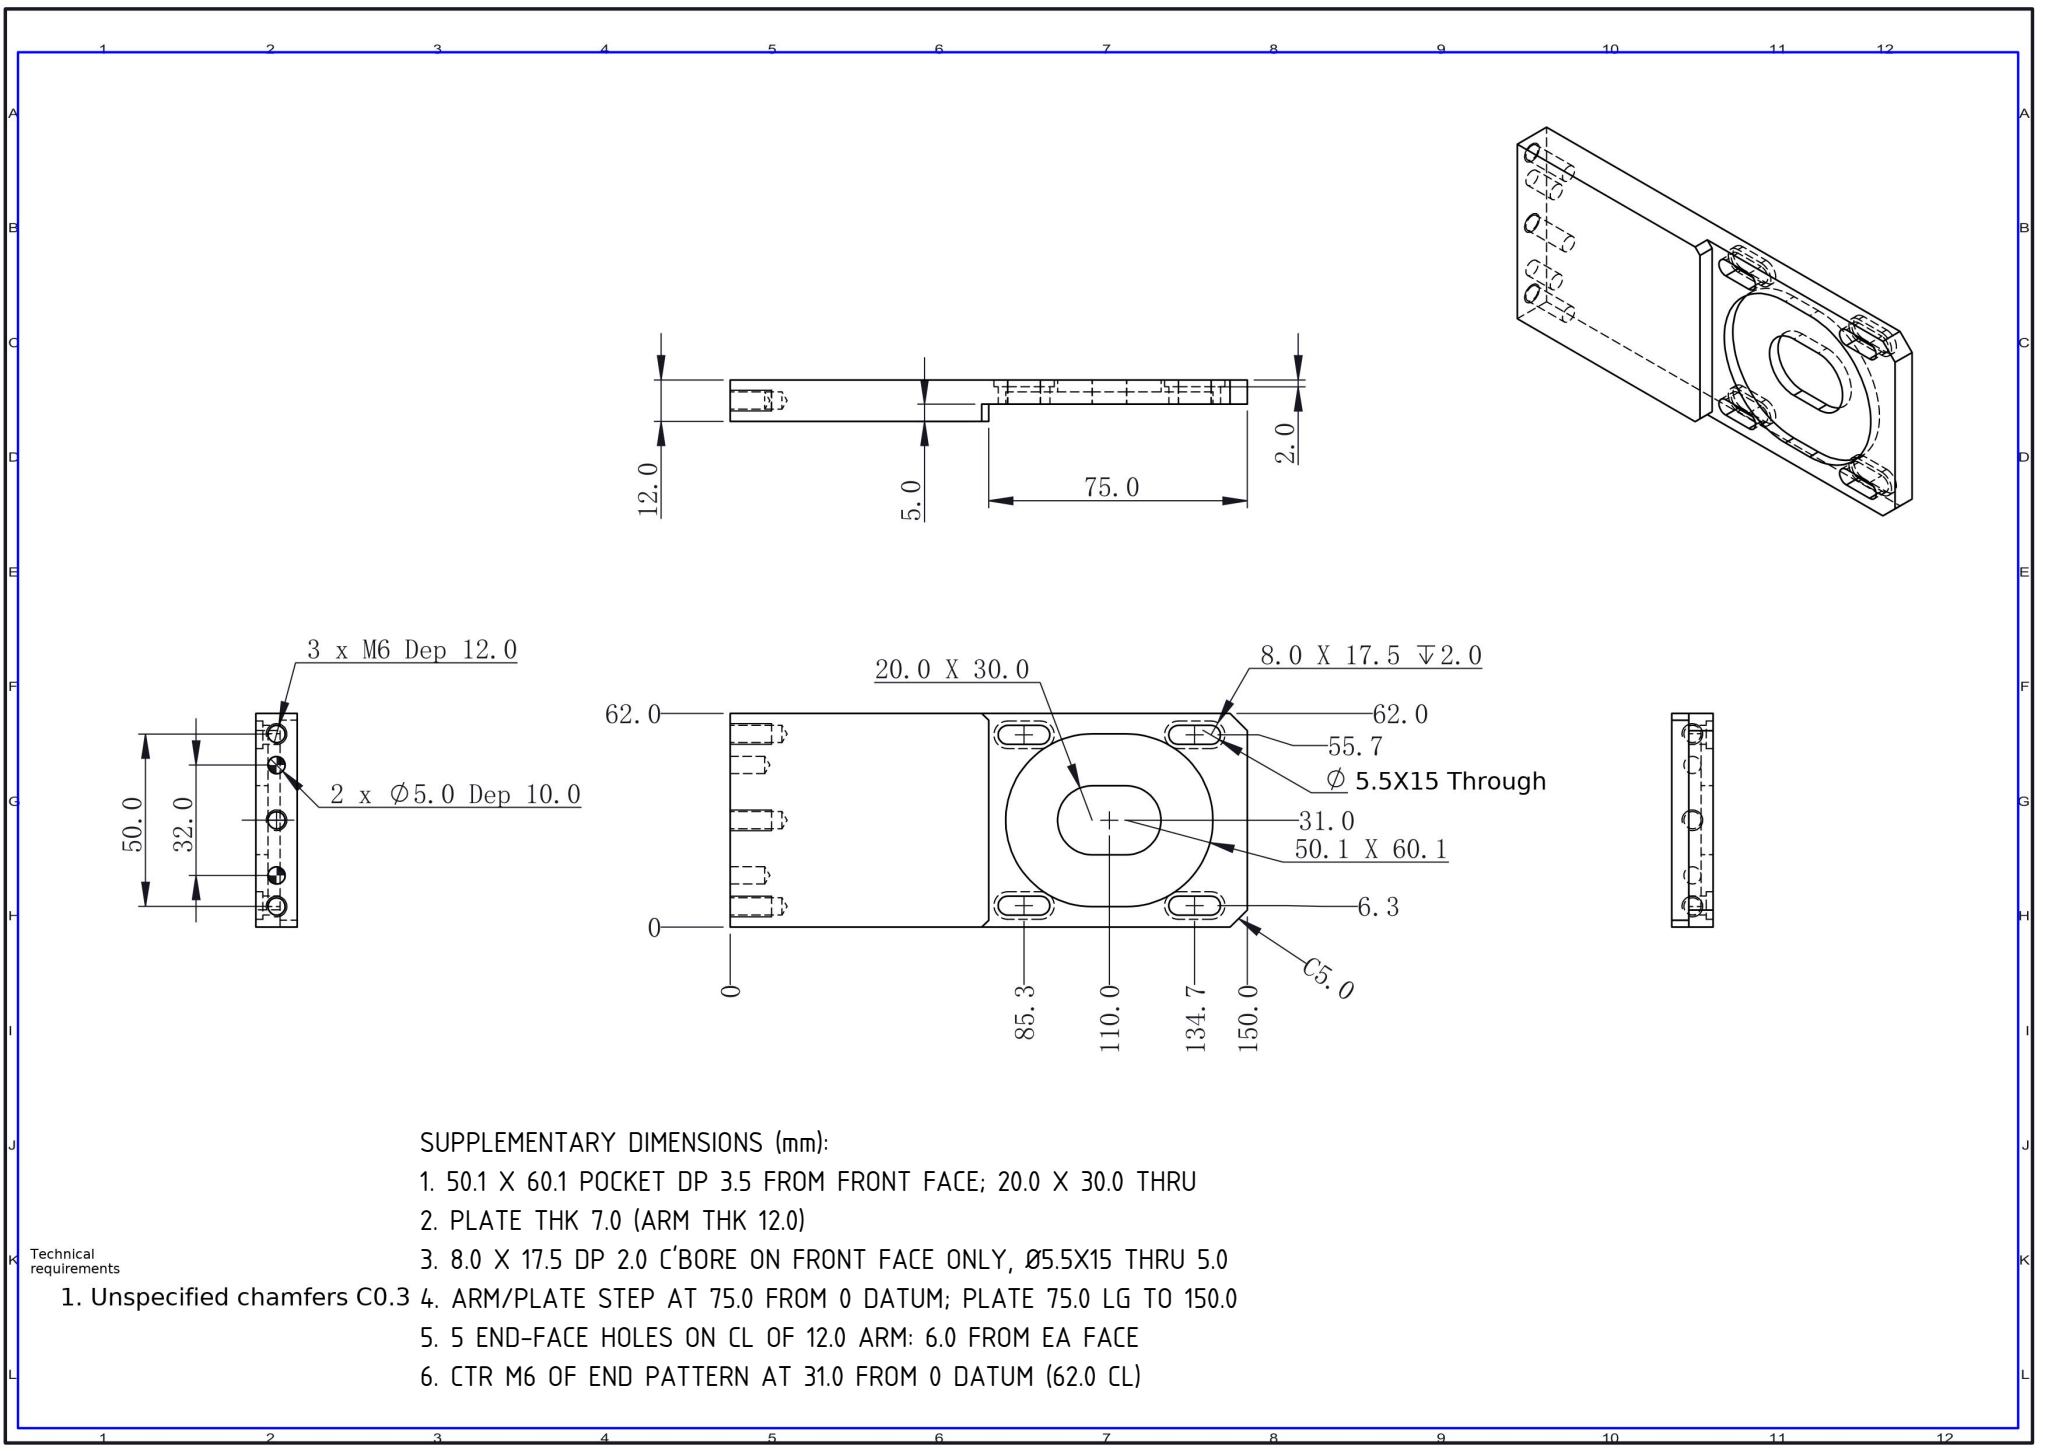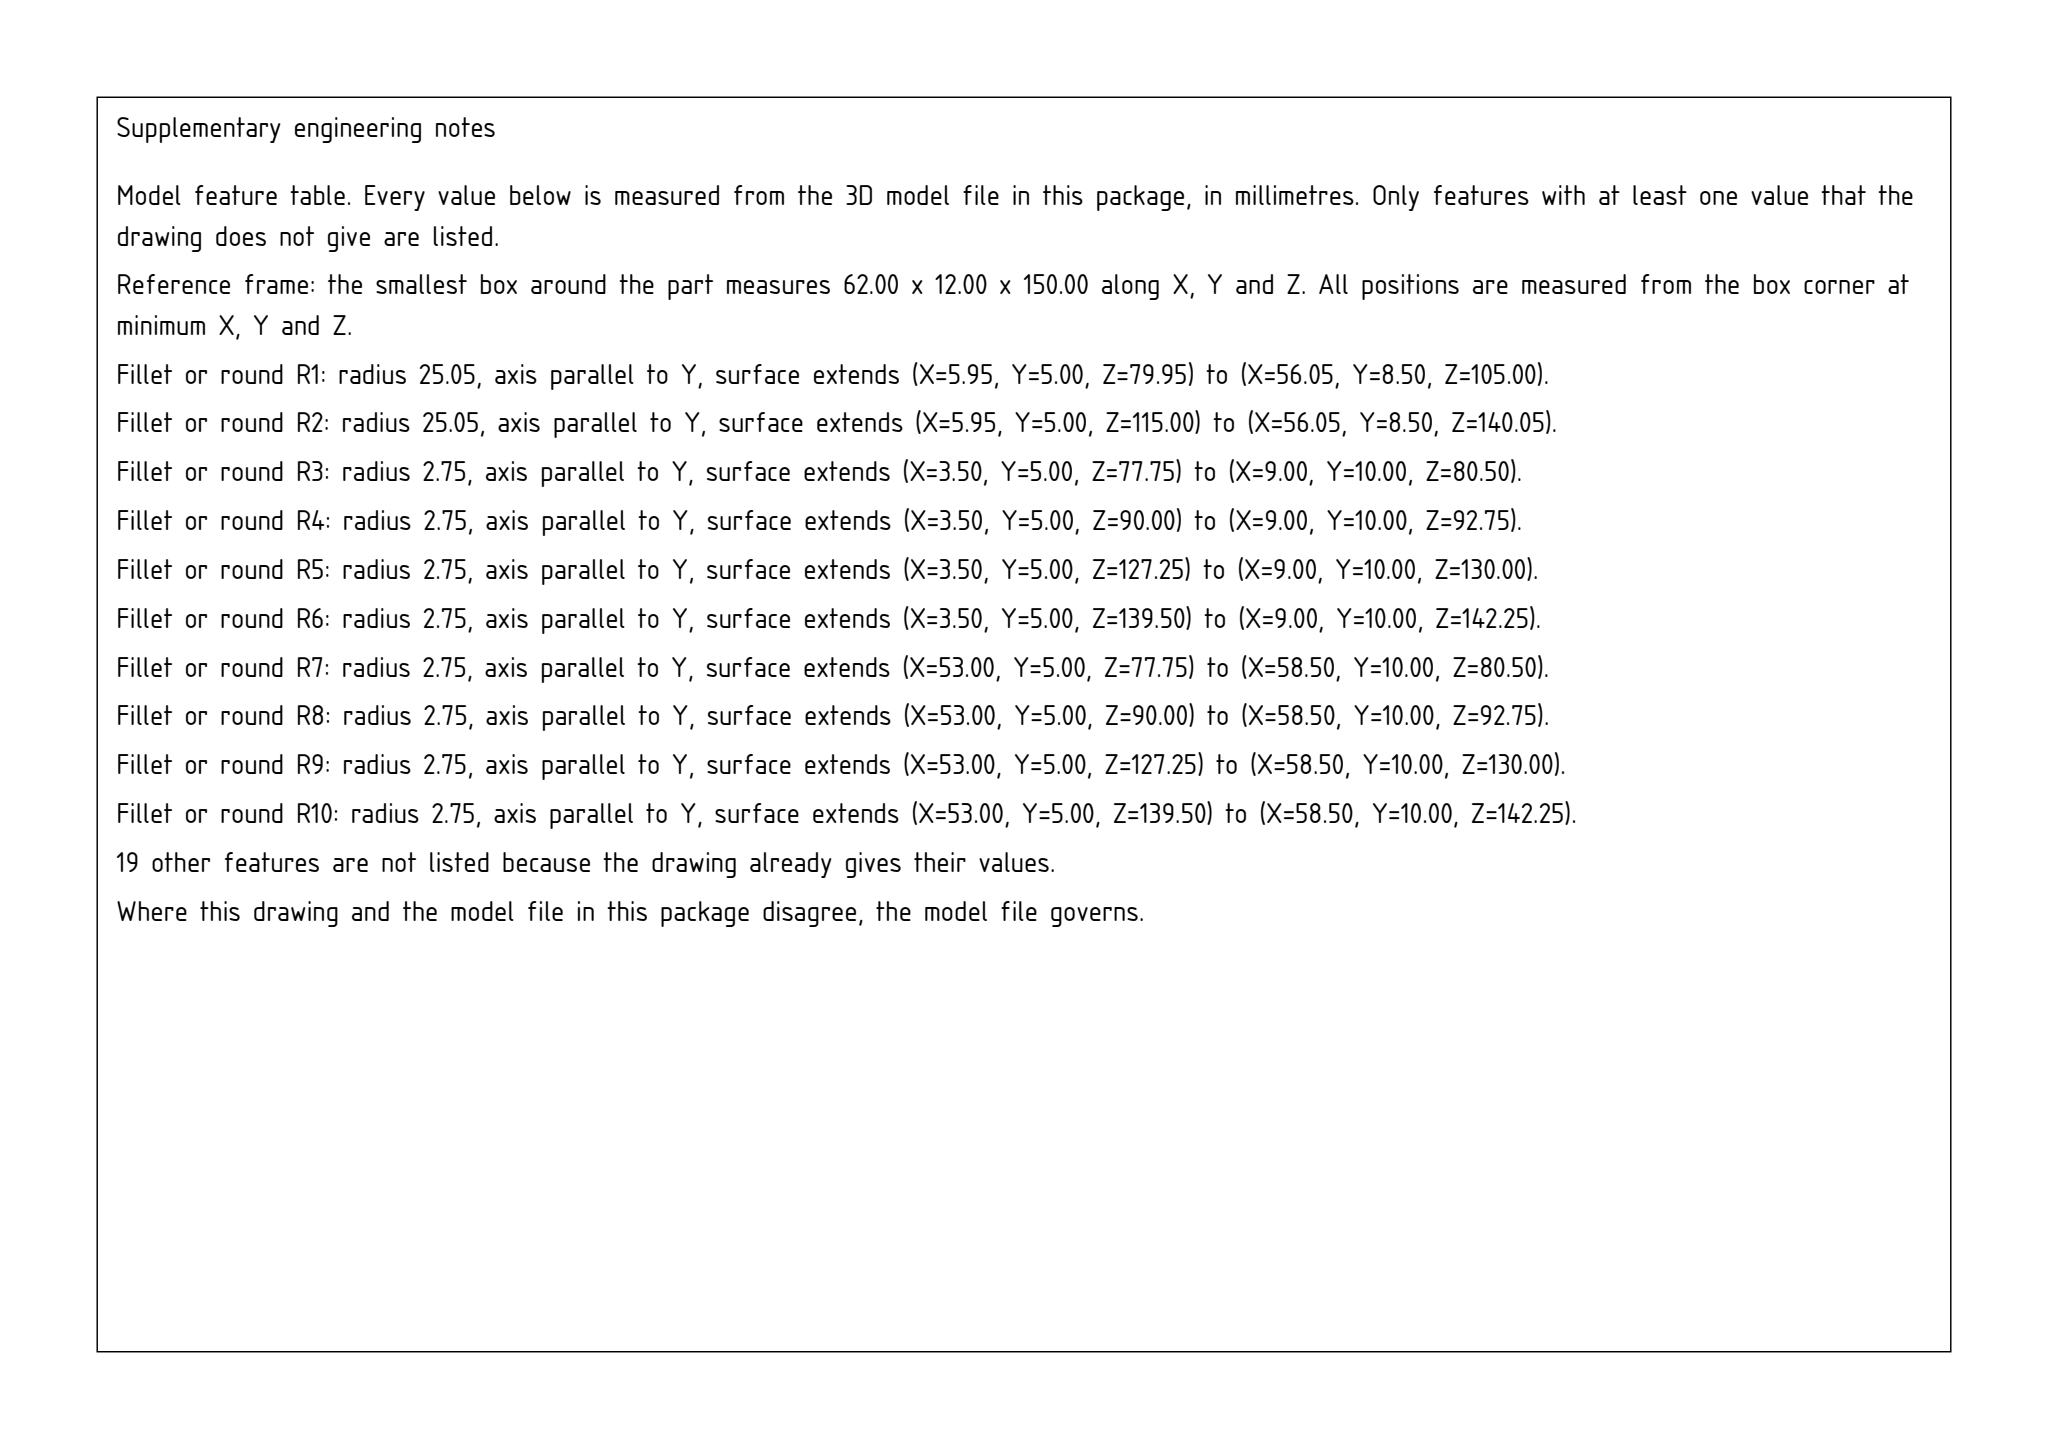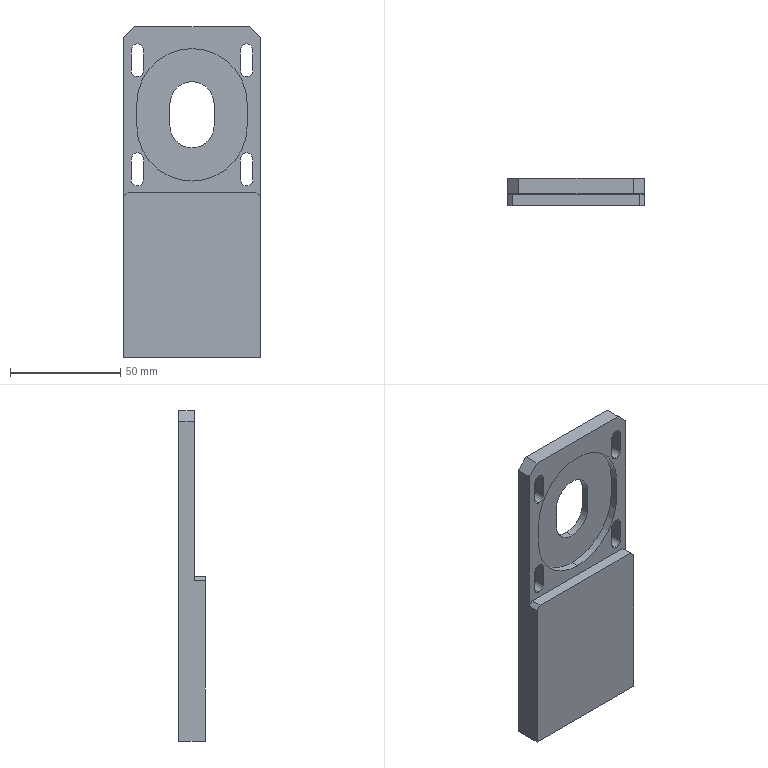Part | SolidWorks | mm | 1 solid | 87 faces | box 62 x 12 x 150 mm | volume 73846 mm3 | cylinder 40 | plane 37 | cone 10 | commonest cylinder face diameters 8 x12 5.5 x12 5 x10 20 x3 50.1 x3